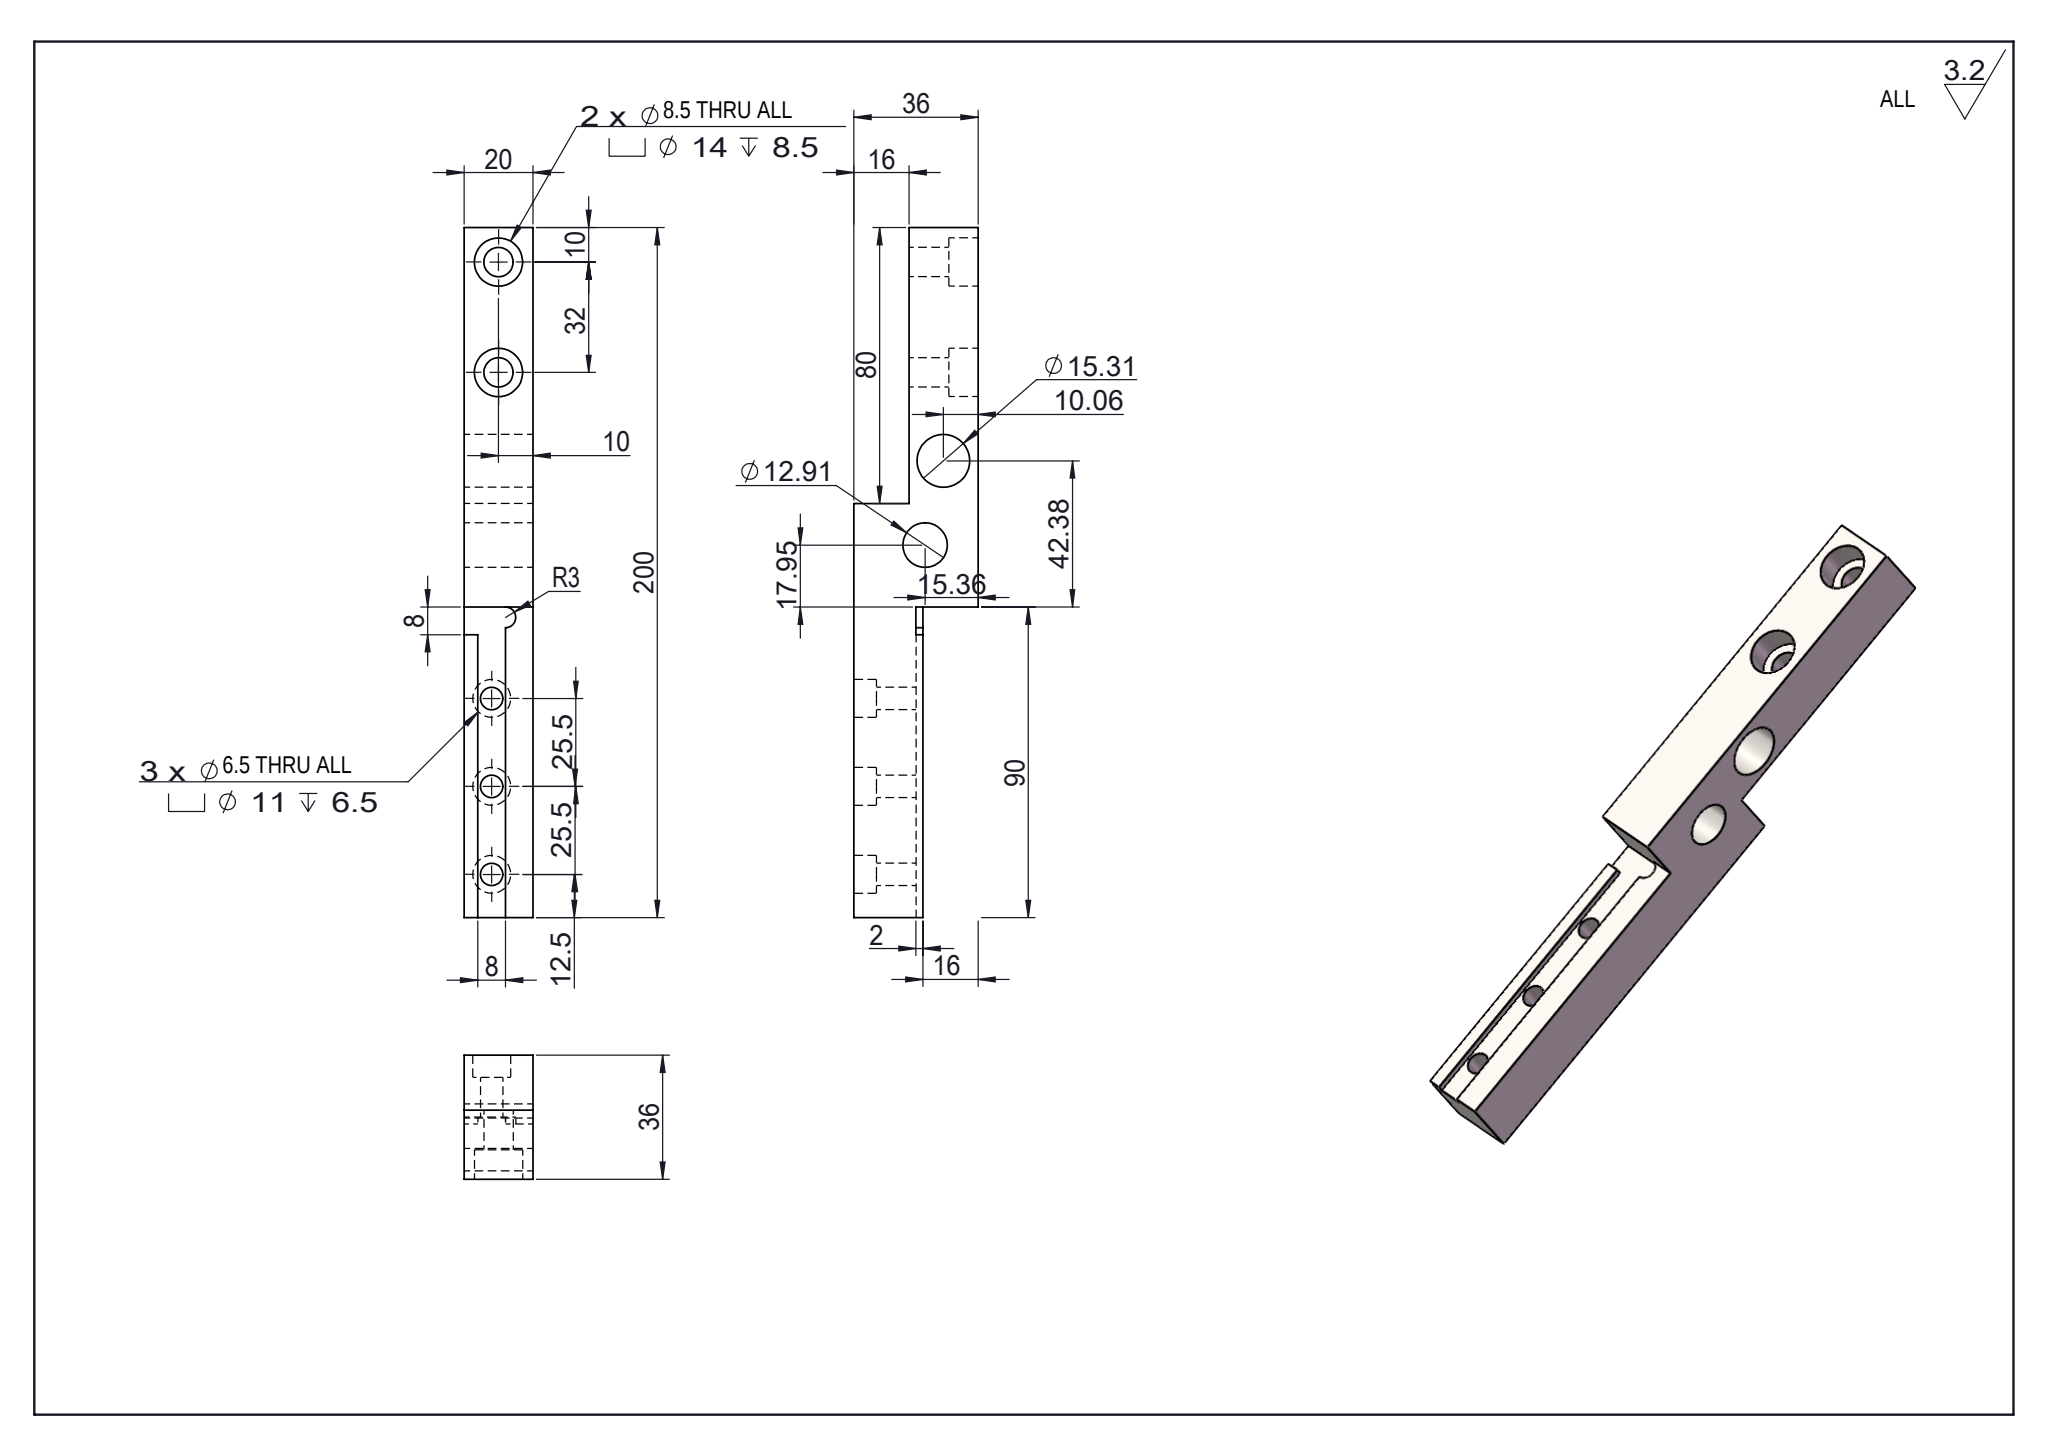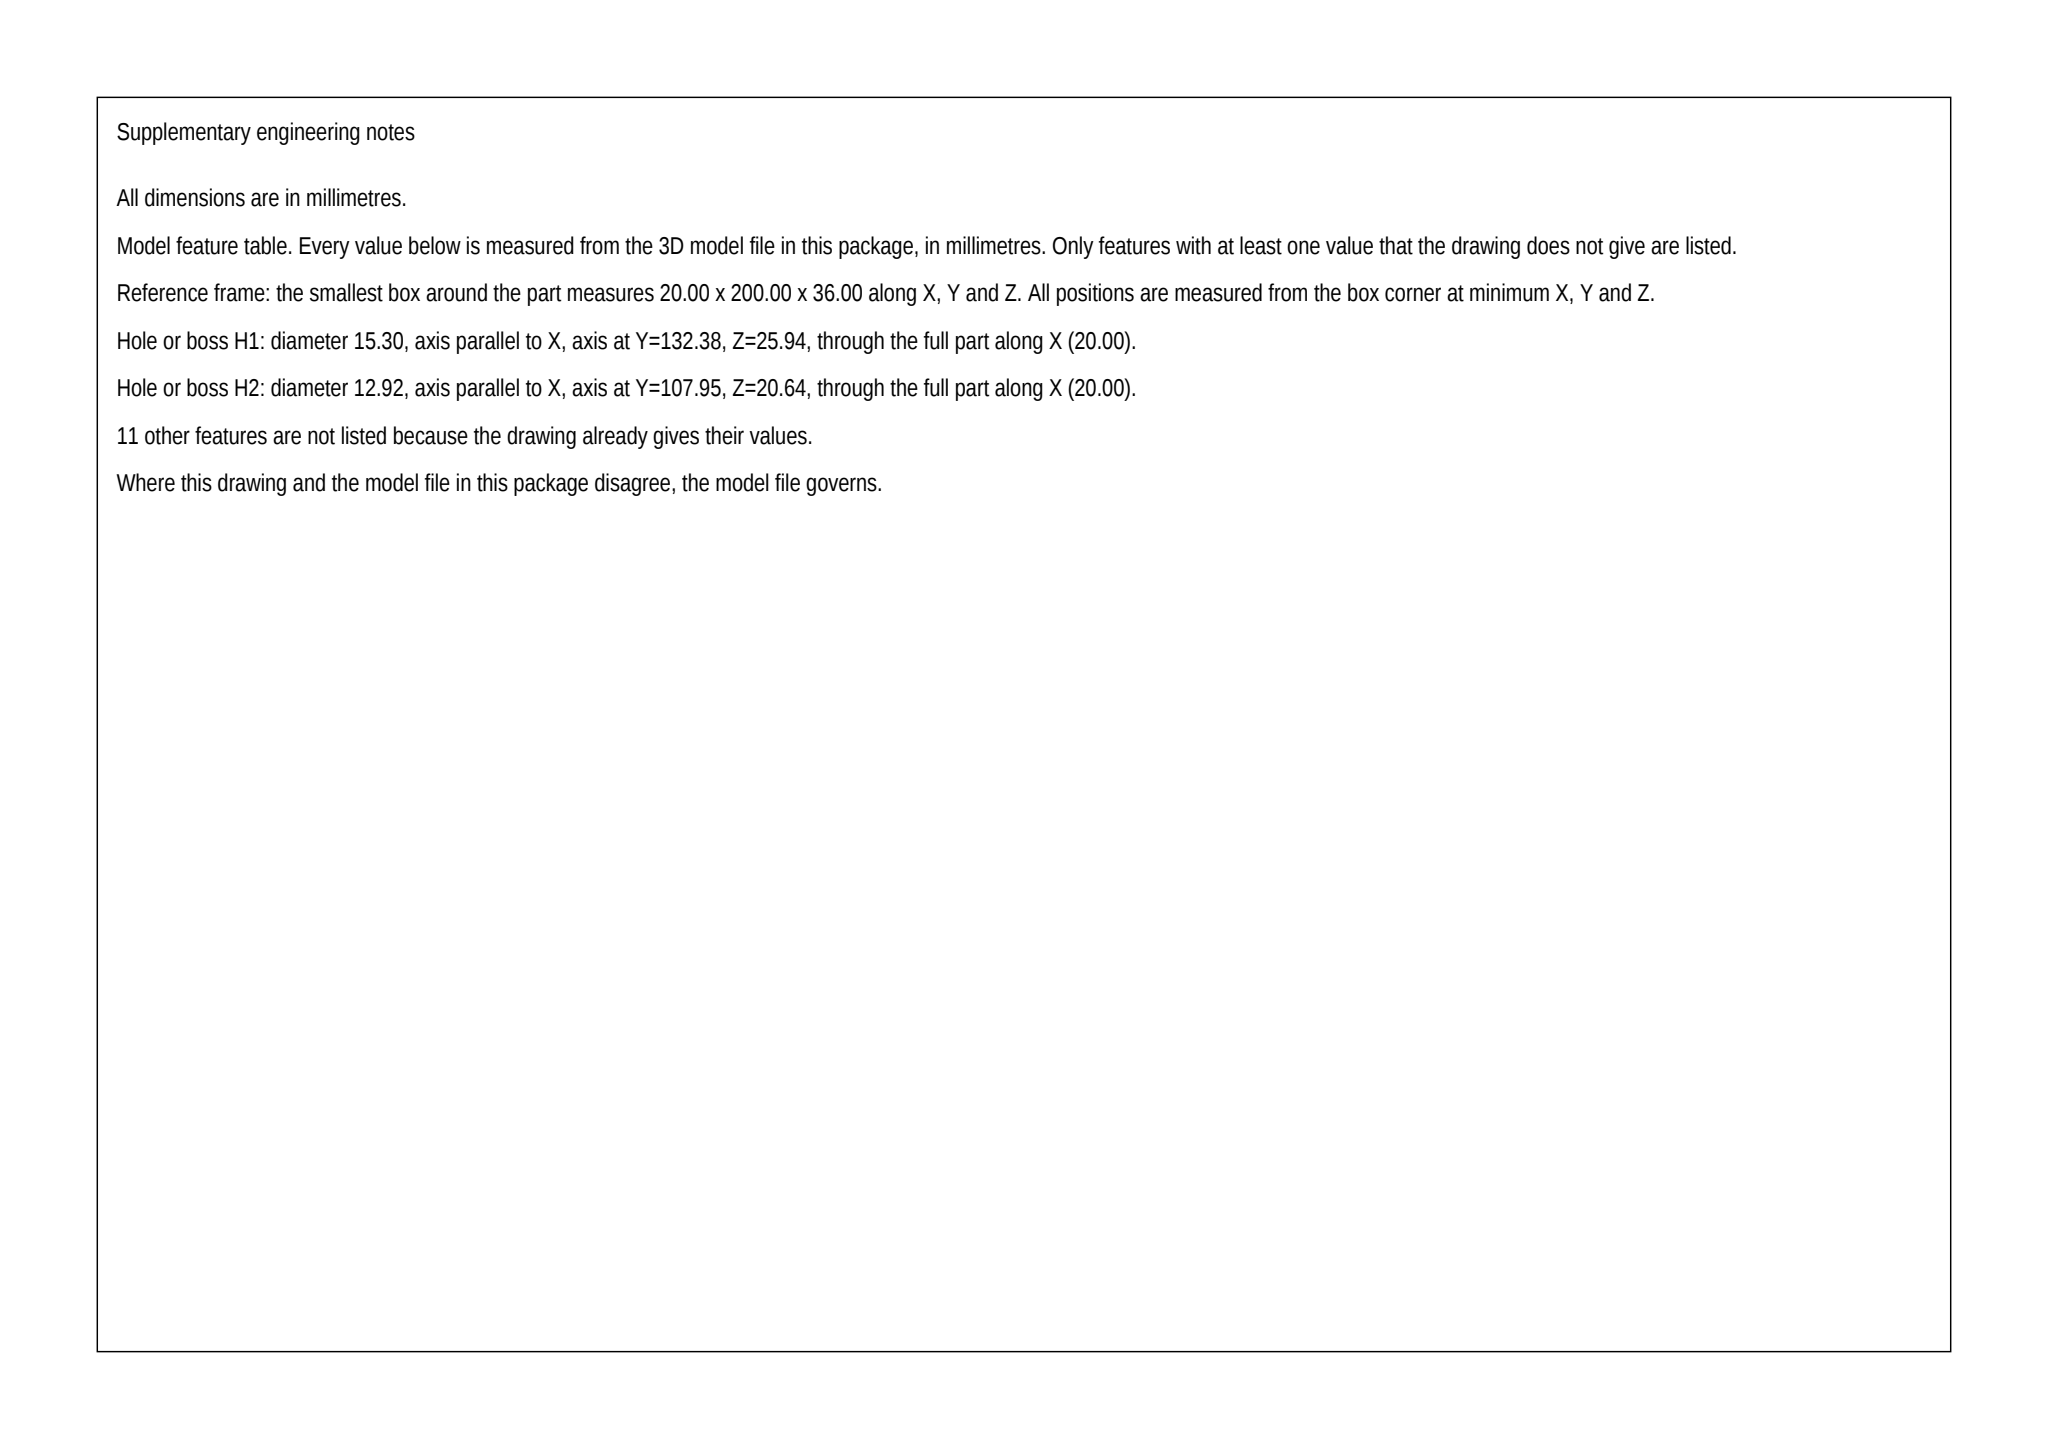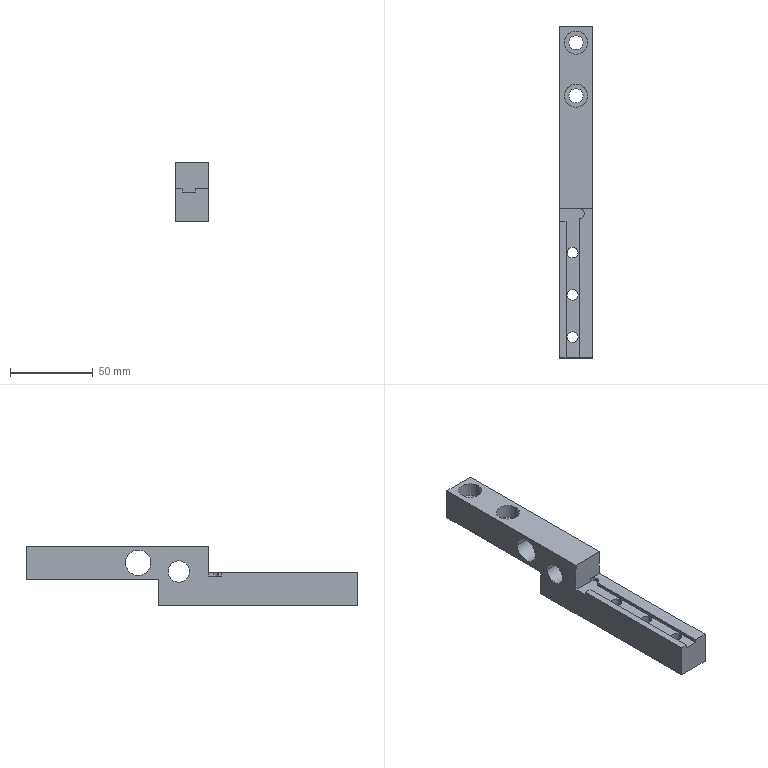Part | SolidWorks | mm | 1 solid | 46 faces | box 20 x 200 x 36 mm | volume 74850 mm3 | cylinder 26 | plane 20 | commonest cylinder face diameters 11 x6 6.5 x6 14 x4 8.5 x4 12.911 x2 15.305 x2 6 x2
build123d program:
from build123d import *

# Parameters (mm, degrees)
SKETCH1_W                                           = 20
SKETCH1_H                                           = 200
BOSS_EXTRUDE1_DEPTH                                 = 36
SKETCH9_W                                           = 16
SKETCH9_H                                           = 90
CUT_EXTRUDE3_DEPTH                                  = 208.525
CUT_EXTRUDE1_DEPTH                                  = 2
CYLINDRICAL_COUNTERSUNK_HOLE_FOR_M8_HEX_D           = 8.5
CYLINDRICAL_COUNTERSUNK_HOLE_FOR_M8_HEX_CBORE_D     = 14
CYLINDRICAL_COUNTERSUNK_HOLE_FOR_M8_HEX_CBORE_DEPTH = 8.5
CYLINDRICAL_COUNTERSUNK_HOLE_FOR_M6_HEX_D           = 6.5
CYLINDRICAL_COUNTERSUNK_HOLE_FOR_M6_HEX_CBORE_D     = 11
CYLINDRICAL_COUNTERSUNK_HOLE_FOR_M6_HEX_CBORE_DEPTH = 6.5
SKETCH8_W                                           = 16
SKETCH8_H                                           = 80
CUT_EXTRUDE2_DEPTH                                  = 208.525
SKETCH10_R                                          = 6.455
SKETCH10_R_2                                        = 7.653
CUT_EXTRUDE4_DEPTH                                  = 80


with BuildPart() as part:
    # Sketch1 → Boss-Extrude1 (new body)
    with BuildSketch(Plane.XY):
        with Locations((157.572, -103.398)):
            Rectangle(SKETCH1_W, SKETCH1_H)
    extrude(amount=BOSS_EXTRUDE1_DEPTH)

    # Sketch9 → Cut-Extrude3 (cut, through all)
    with BuildSketch(Plane(origin=(167.572, 0, 0), x_dir=(0, 0, -1), z_dir=(1, 0, 0))):
        with Locations((-28, -158.398)):
            Rectangle(SKETCH9_W, SKETCH9_H)
    extrude(amount=-CUT_EXTRUDE3_DEPTH, mode=Mode.SUBTRACT)

    # Sketch2 → Cut-Extrude1 (cut)
    with BuildSketch(Plane.XY.offset(20)):
        with BuildLine():
            Line((151.572, -121.398), (137.572, -121.398))
            Line((137.572, -121.398), (137.572, -113.398))
            Line((137.572, -113.398), (159.572, -113.398))
            ThreePointArc((159.572, -113.398), (162.572, -116.398), (159.572, -119.398))
            Line((159.572, -119.398), (159.572, -365.398))
            Line((159.572, -365.398), (151.572, -365.398))
            Line((151.572, -365.398), (151.572, -121.398))
        make_face()
    extrude(amount=-CUT_EXTRUDE1_DEPTH, mode=Mode.SUBTRACT)

    # Cylindrical Countersunk Hole for M8 Hex (through all)
    with Locations(Plane.XY.offset(36)):
        with Locations((157.572, -13.398), (157.572, -45.398)):
            CounterBoreHole(CYLINDRICAL_COUNTERSUNK_HOLE_FOR_M8_HEX_D / 2, CYLINDRICAL_COUNTERSUNK_HOLE_FOR_M8_HEX_CBORE_D / 2, CYLINDRICAL_COUNTERSUNK_HOLE_FOR_M8_HEX_CBORE_DEPTH)

    # Cylindrical Countersunk Hole for M6 Hex (through all)
    with Locations(Plane(origin=(0, 0, 0), x_dir=(-1, 0, 0), z_dir=(0, 0, -1))):
        with Locations((-155.572, -139.898), (-155.572, -165.398), (-155.572, -190.898)):
            CounterBoreHole(CYLINDRICAL_COUNTERSUNK_HOLE_FOR_M6_HEX_D / 2, CYLINDRICAL_COUNTERSUNK_HOLE_FOR_M6_HEX_CBORE_D / 2, CYLINDRICAL_COUNTERSUNK_HOLE_FOR_M6_HEX_CBORE_DEPTH)

    # Sketch8 → Cut-Extrude2 (cut, through all)
    with BuildSketch(Plane(origin=(167.572, 0, 0), x_dir=(0, 0, -1), z_dir=(1, 0, 0))):
        with Locations((-8, -43.398)):
            Rectangle(SKETCH8_W, SKETCH8_H)
    extrude(amount=-CUT_EXTRUDE2_DEPTH, mode=Mode.SUBTRACT)

    # Sketch10 → Cut-Extrude4 (cut)
    with BuildSketch(Plane(origin=(167.572, 0, 0), x_dir=(0, 0, -1), z_dir=(1, 0, 0))):
        with Locations(Location((-20.642, -95.451, 0), (0, 0, 90))):
            Circle(SKETCH10_R)
        with Locations(Location((-25.94, -71.021, 0), (0, 0, 90))):
            Circle(SKETCH10_R_2)
    extrude(amount=-CUT_EXTRUDE4_DEPTH, mode=Mode.SUBTRACT)


solid = part.part